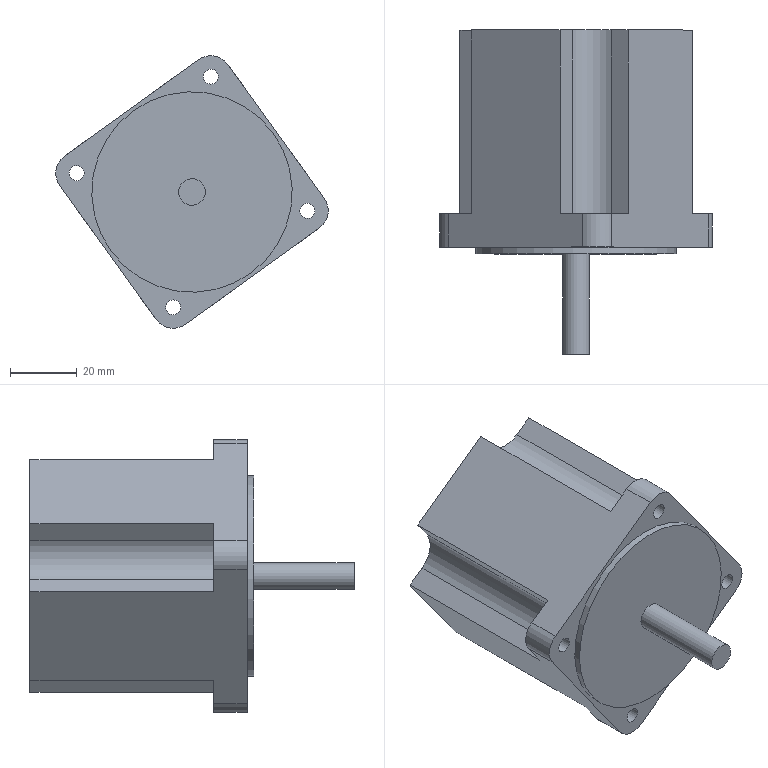Component | NX | MOTOR | 1 solid | 34 faces | volume 212475 mm3 | plane 20 | cylinder 14 | commonest cylinder face diameters 12.503 x4 16.688 x4 4.5 x4 8 x1 60 x1